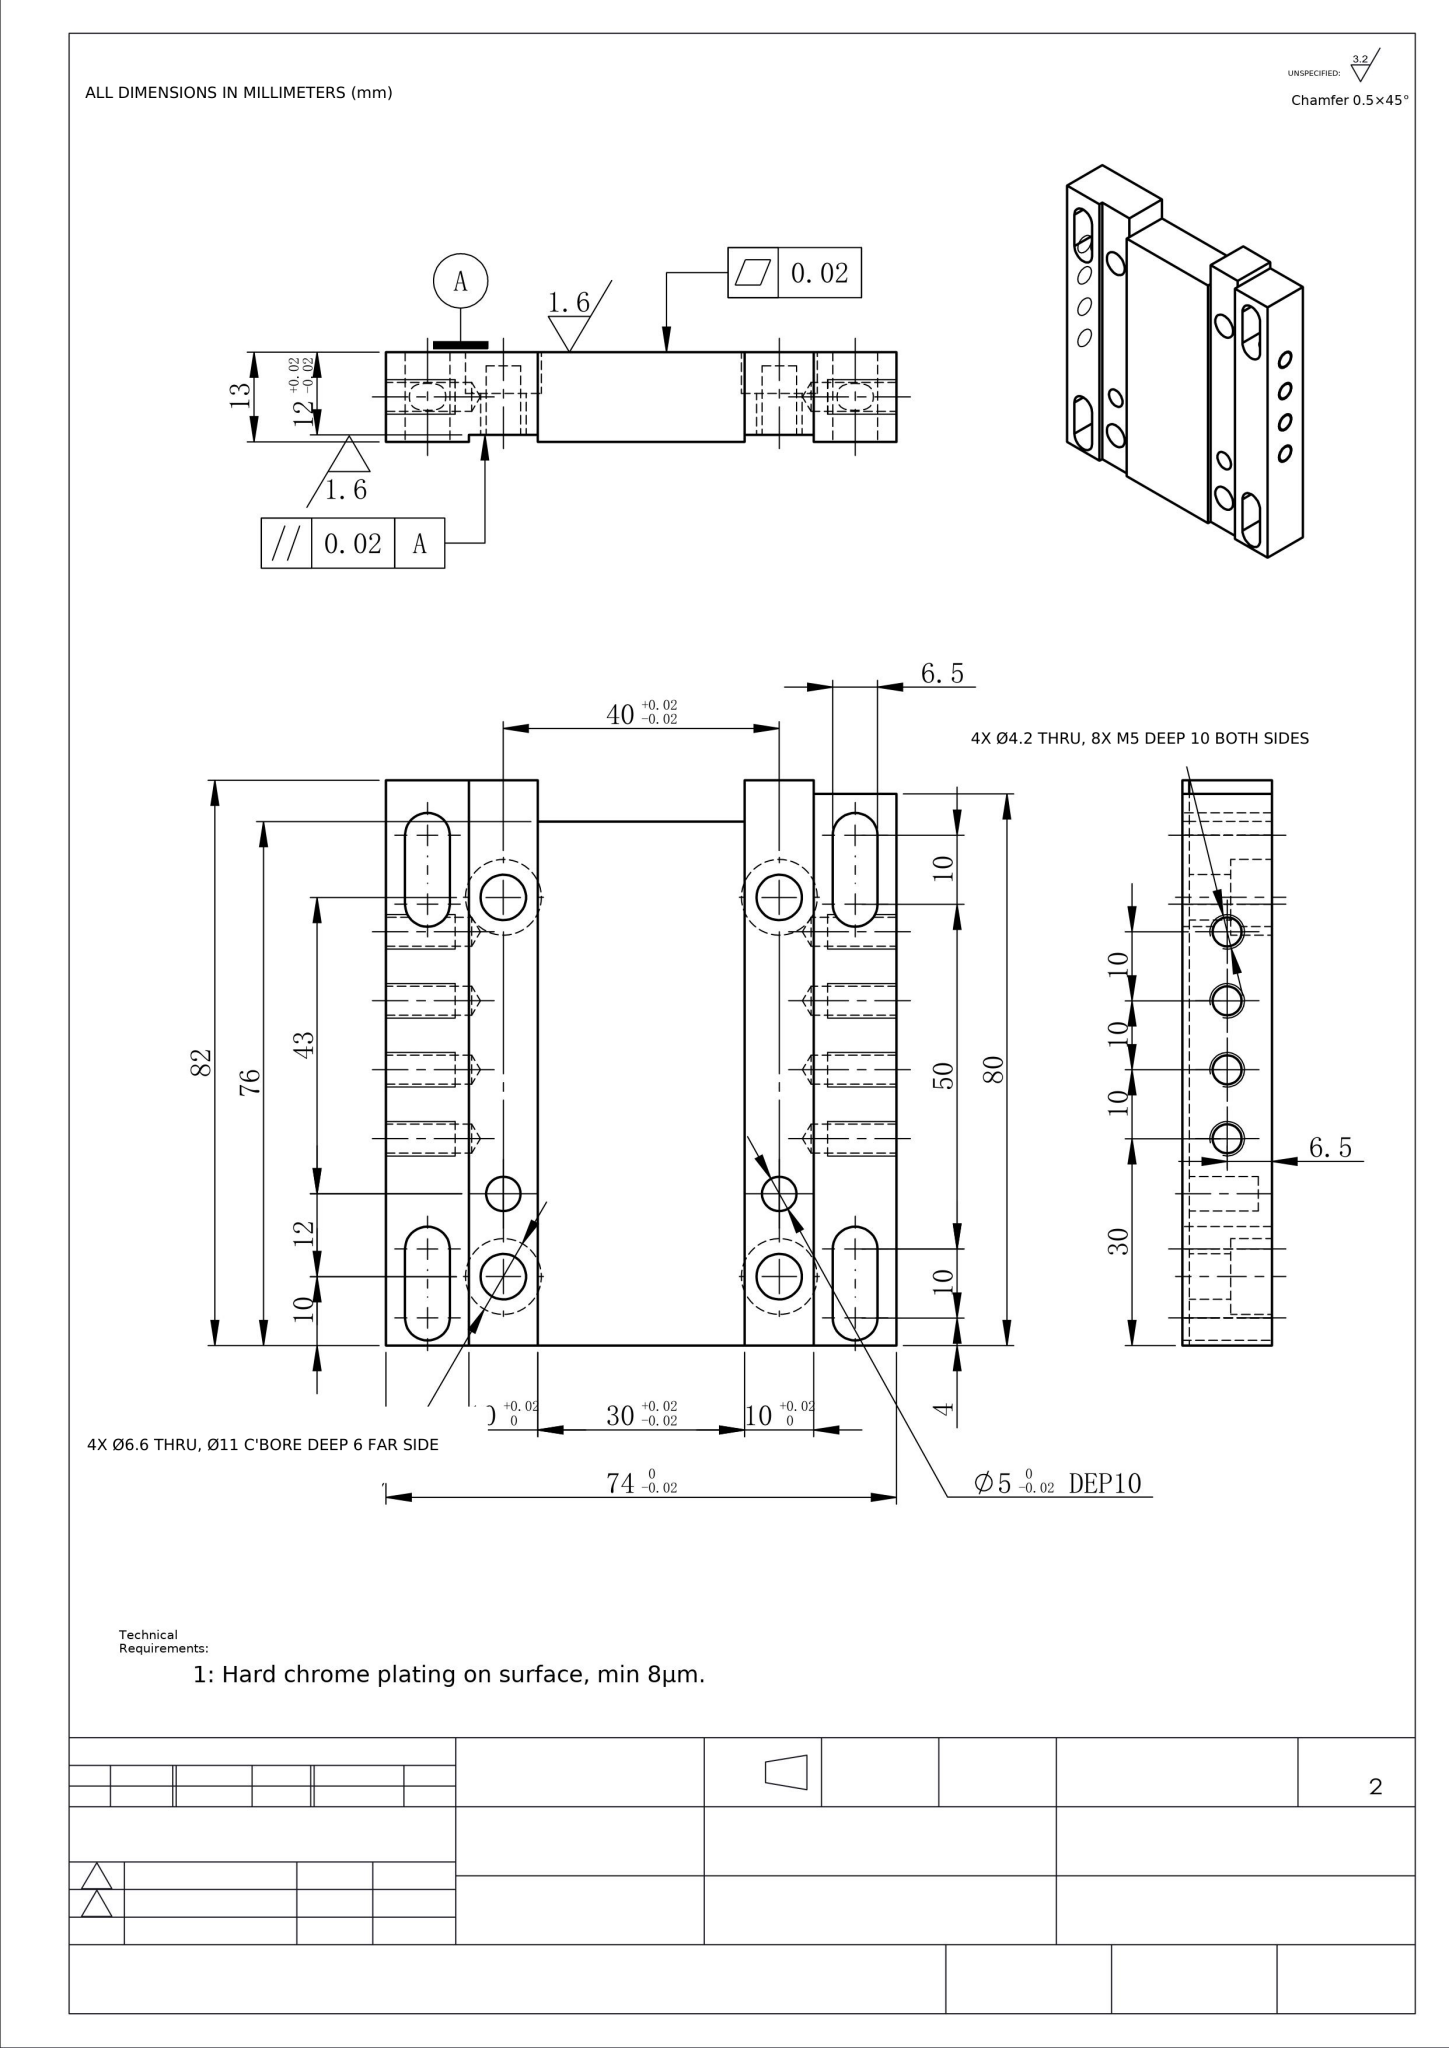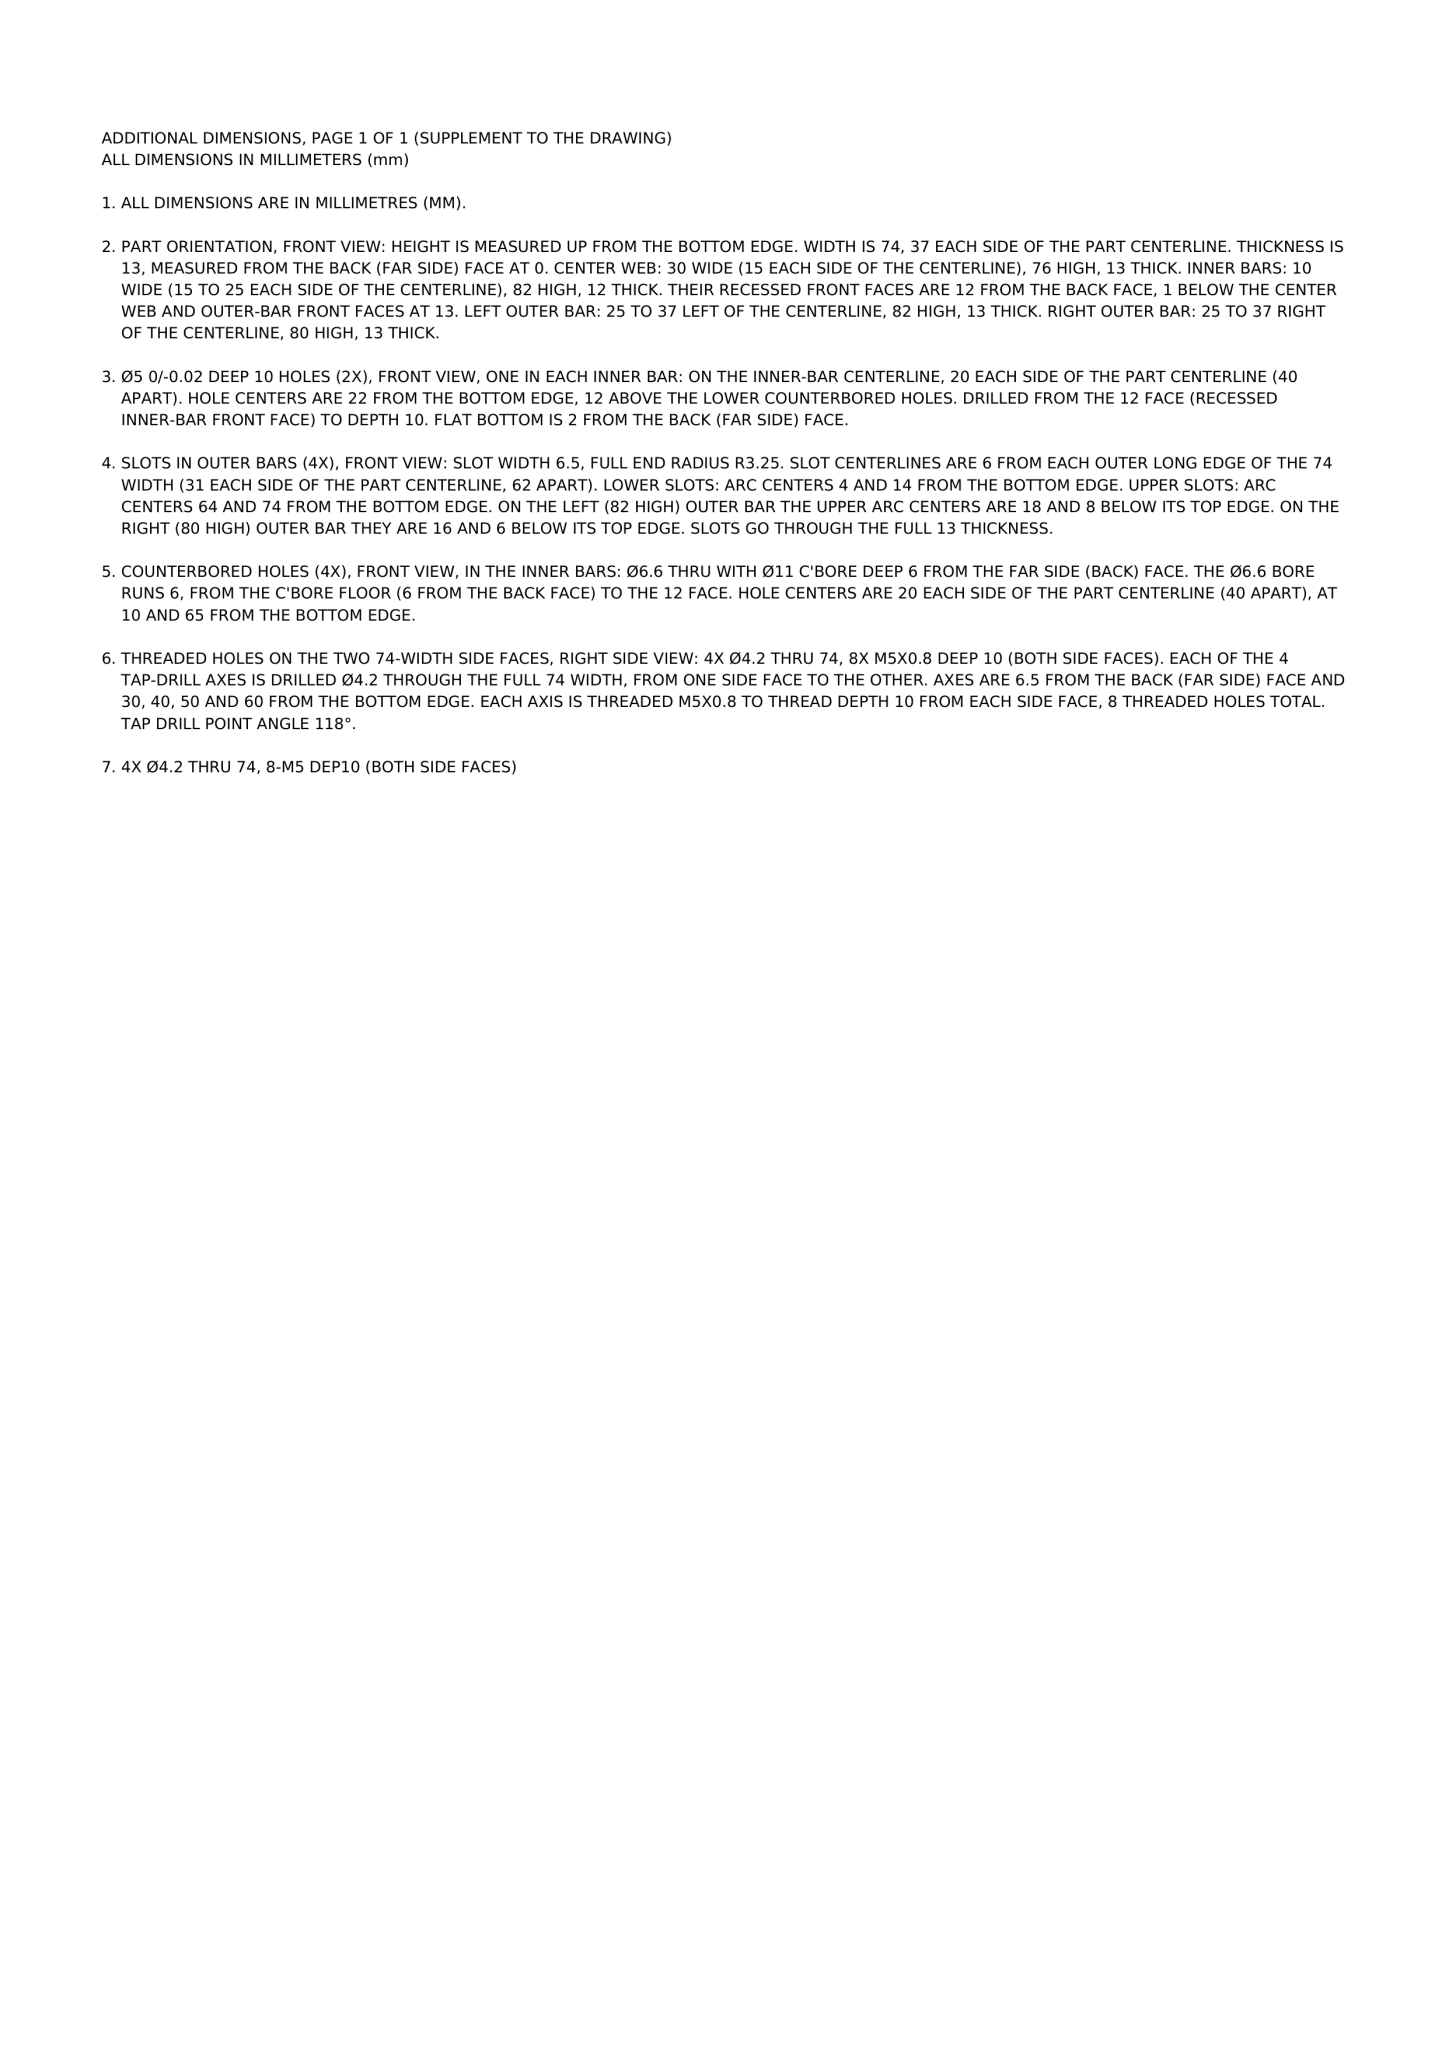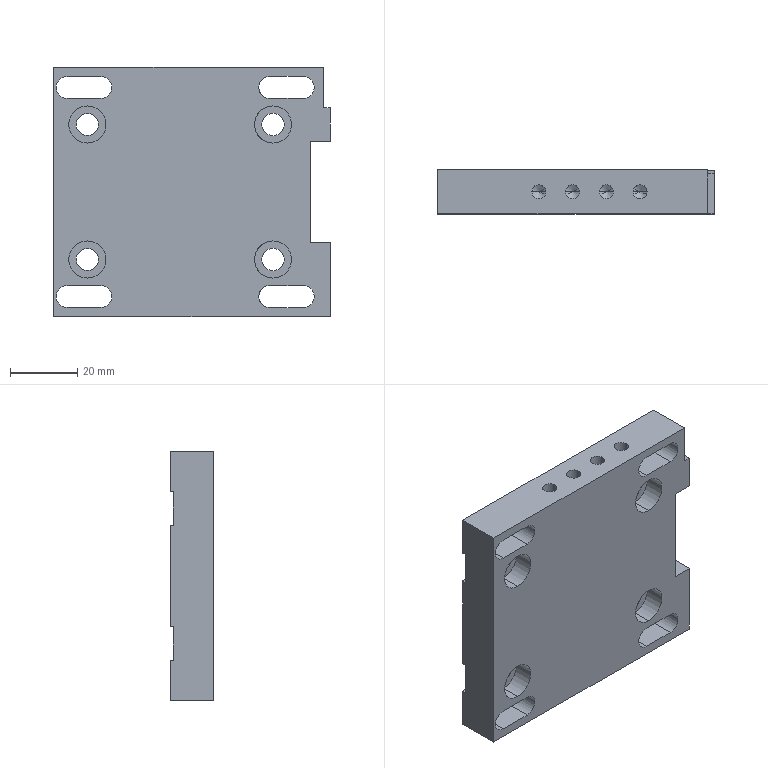Part | NX | mm | 1 solid | 94 faces | box 82 x 13 x 74 mm | volume 64597 mm3 | cylinder 44 | plane 34 | cone 16 | commonest cylinder face diameters 4.2 x16 11 x8 6.6 x8 6.5 x8 5 x4